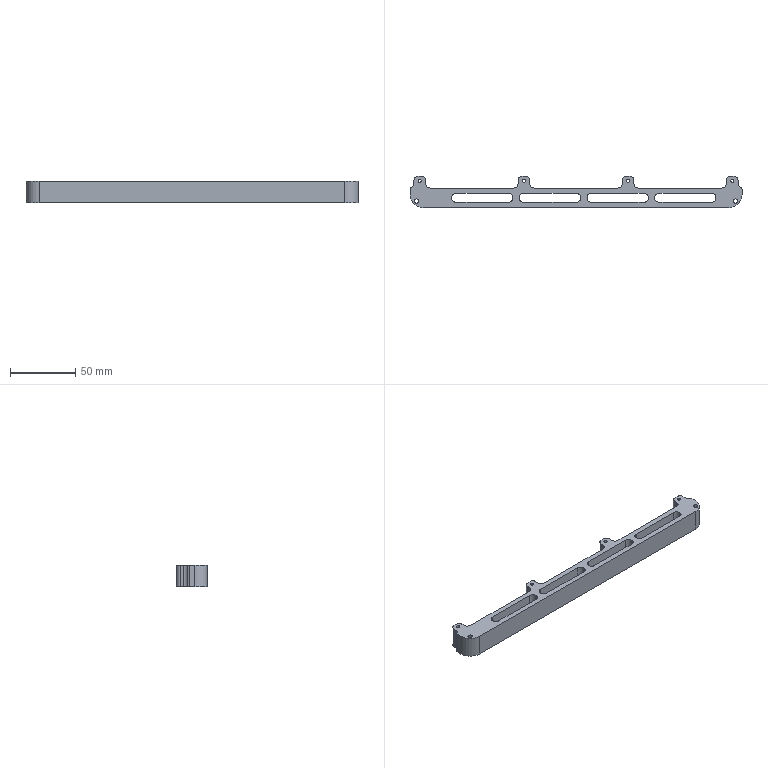CAM job | Mastercam | mm | 11 operations | part box 255 x 24 x 16.7
1. Facing | 24 - 100 平铣刀
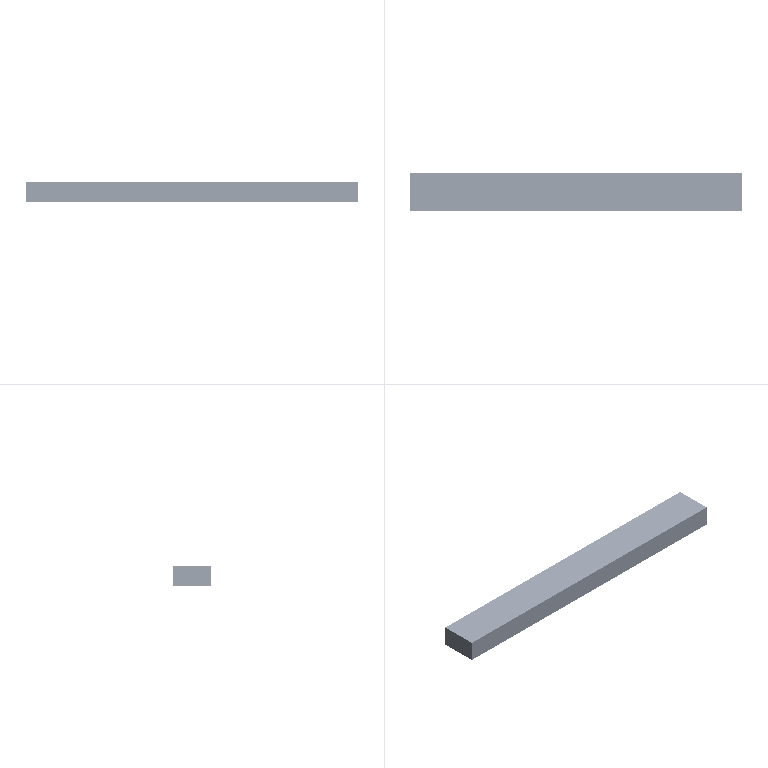2. 2D High Speed (2D Dynamic Mill) | 10 - 10 平铣刀
3. Contour (Remachining) | 6 - 6 平铣刀
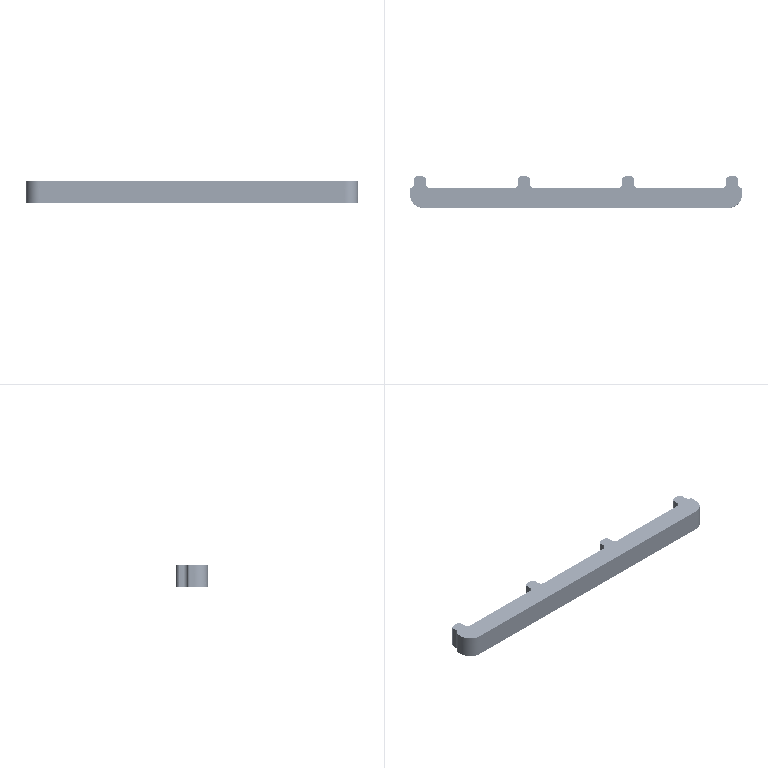4. Contour (Ramp) | 6 - 6 平铣刀
5. Contour (2D) | 6 - 6 平铣刀
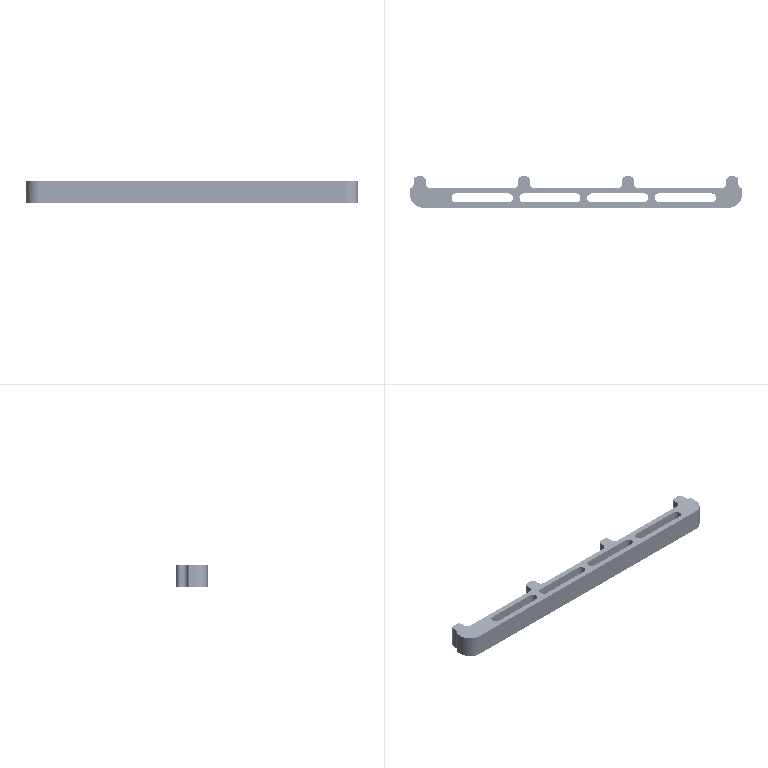6. Contour (Ramp) | 6 - 6 平铣刀
7. Drill/Counterbore | 7 - 4 倒角刀
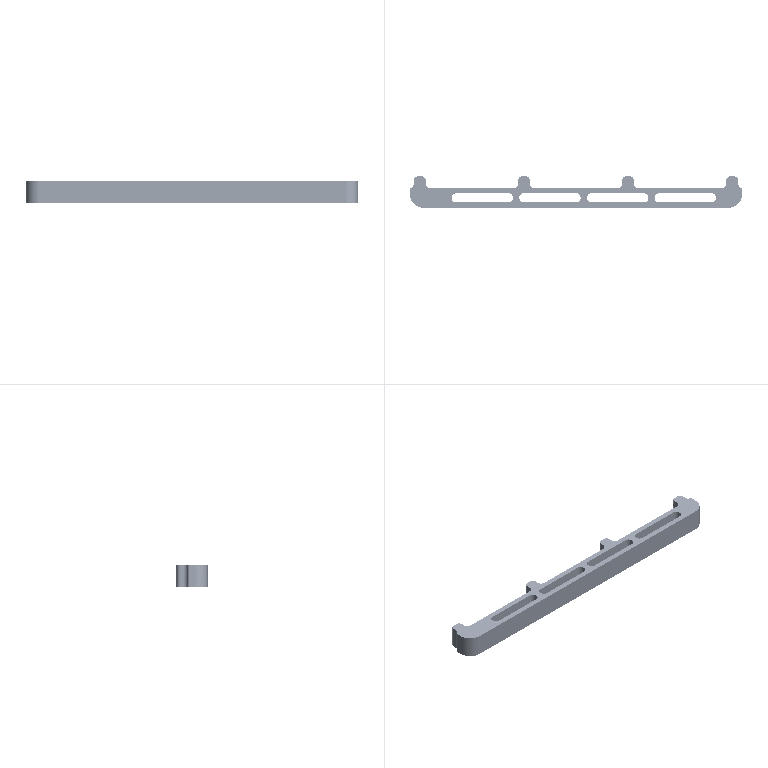8. Contour (2D chamfer) | 7 - 4 倒角刀
9. Facing | 10 - 10 平铣刀
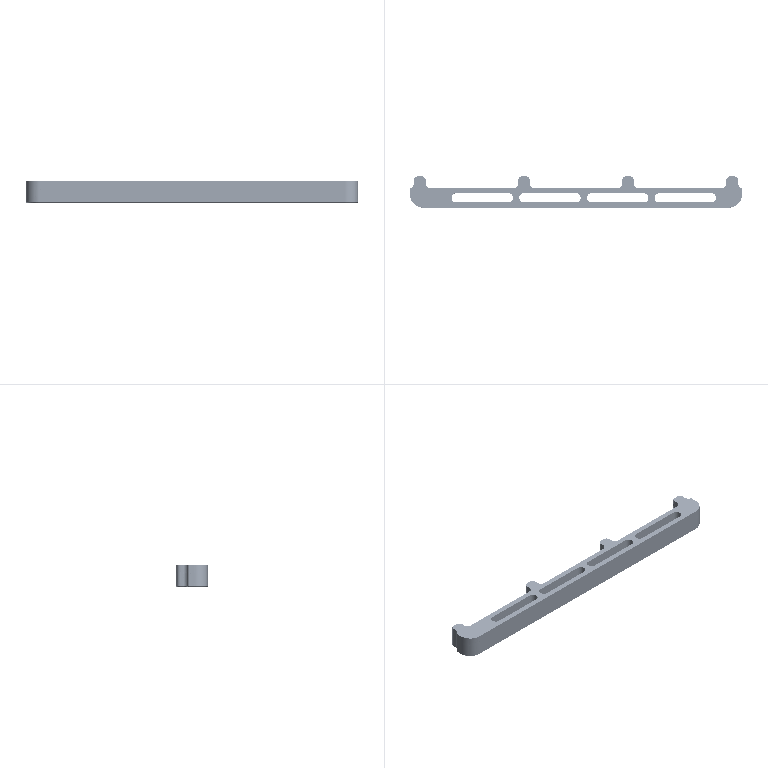10. Facing | 10 - 10 平铣刀
11. Contour (2D chamfer) | 7 - 4 倒角刀